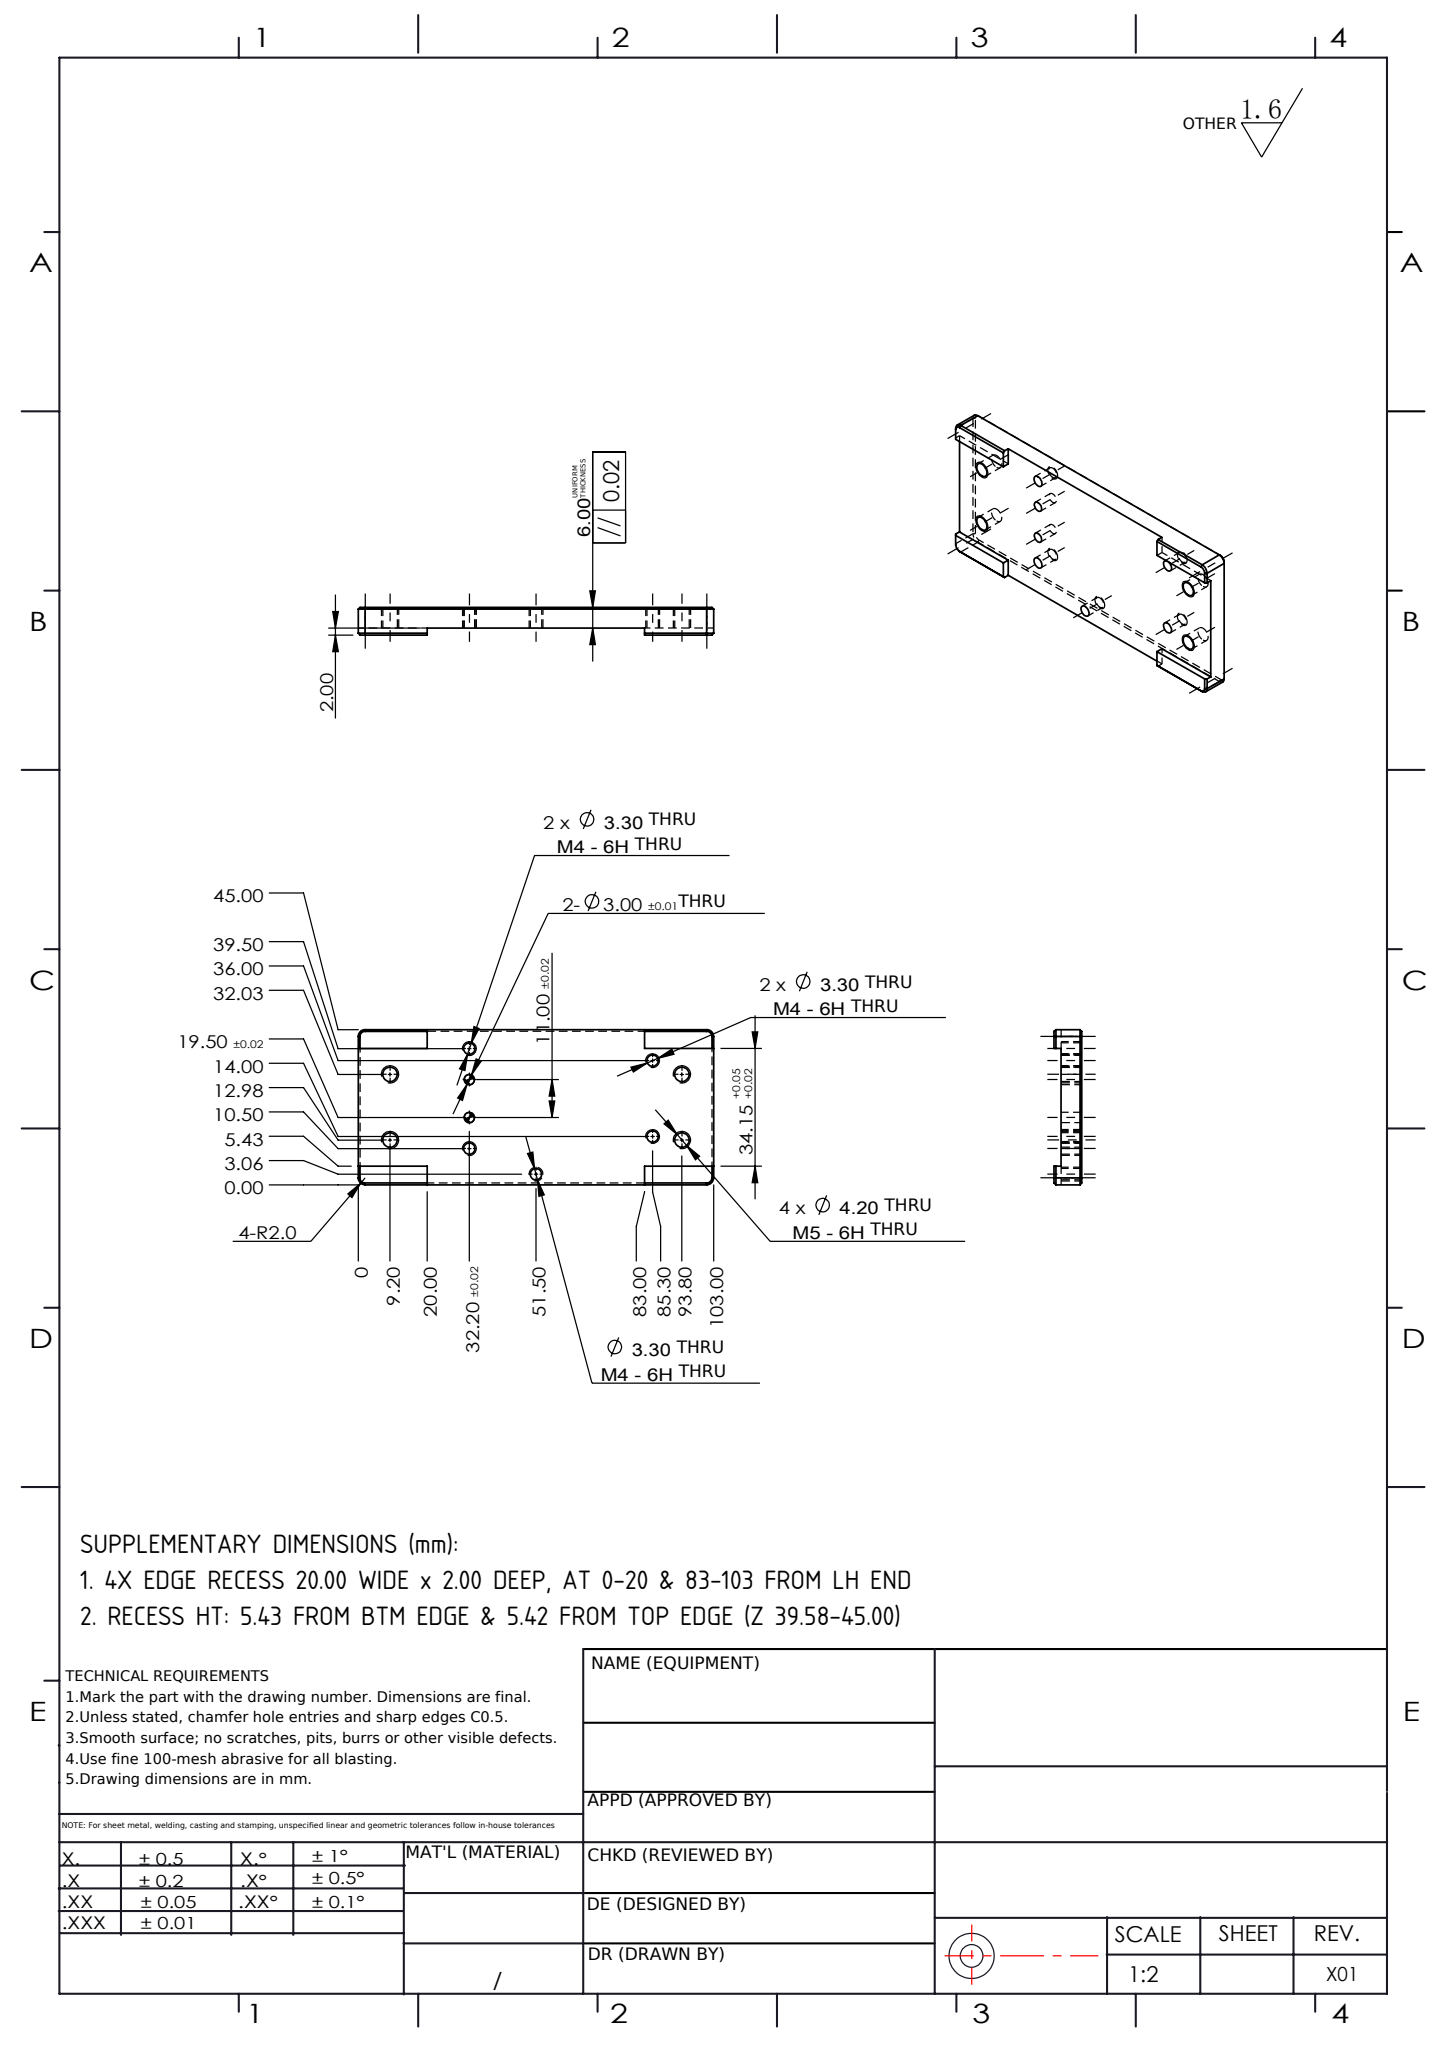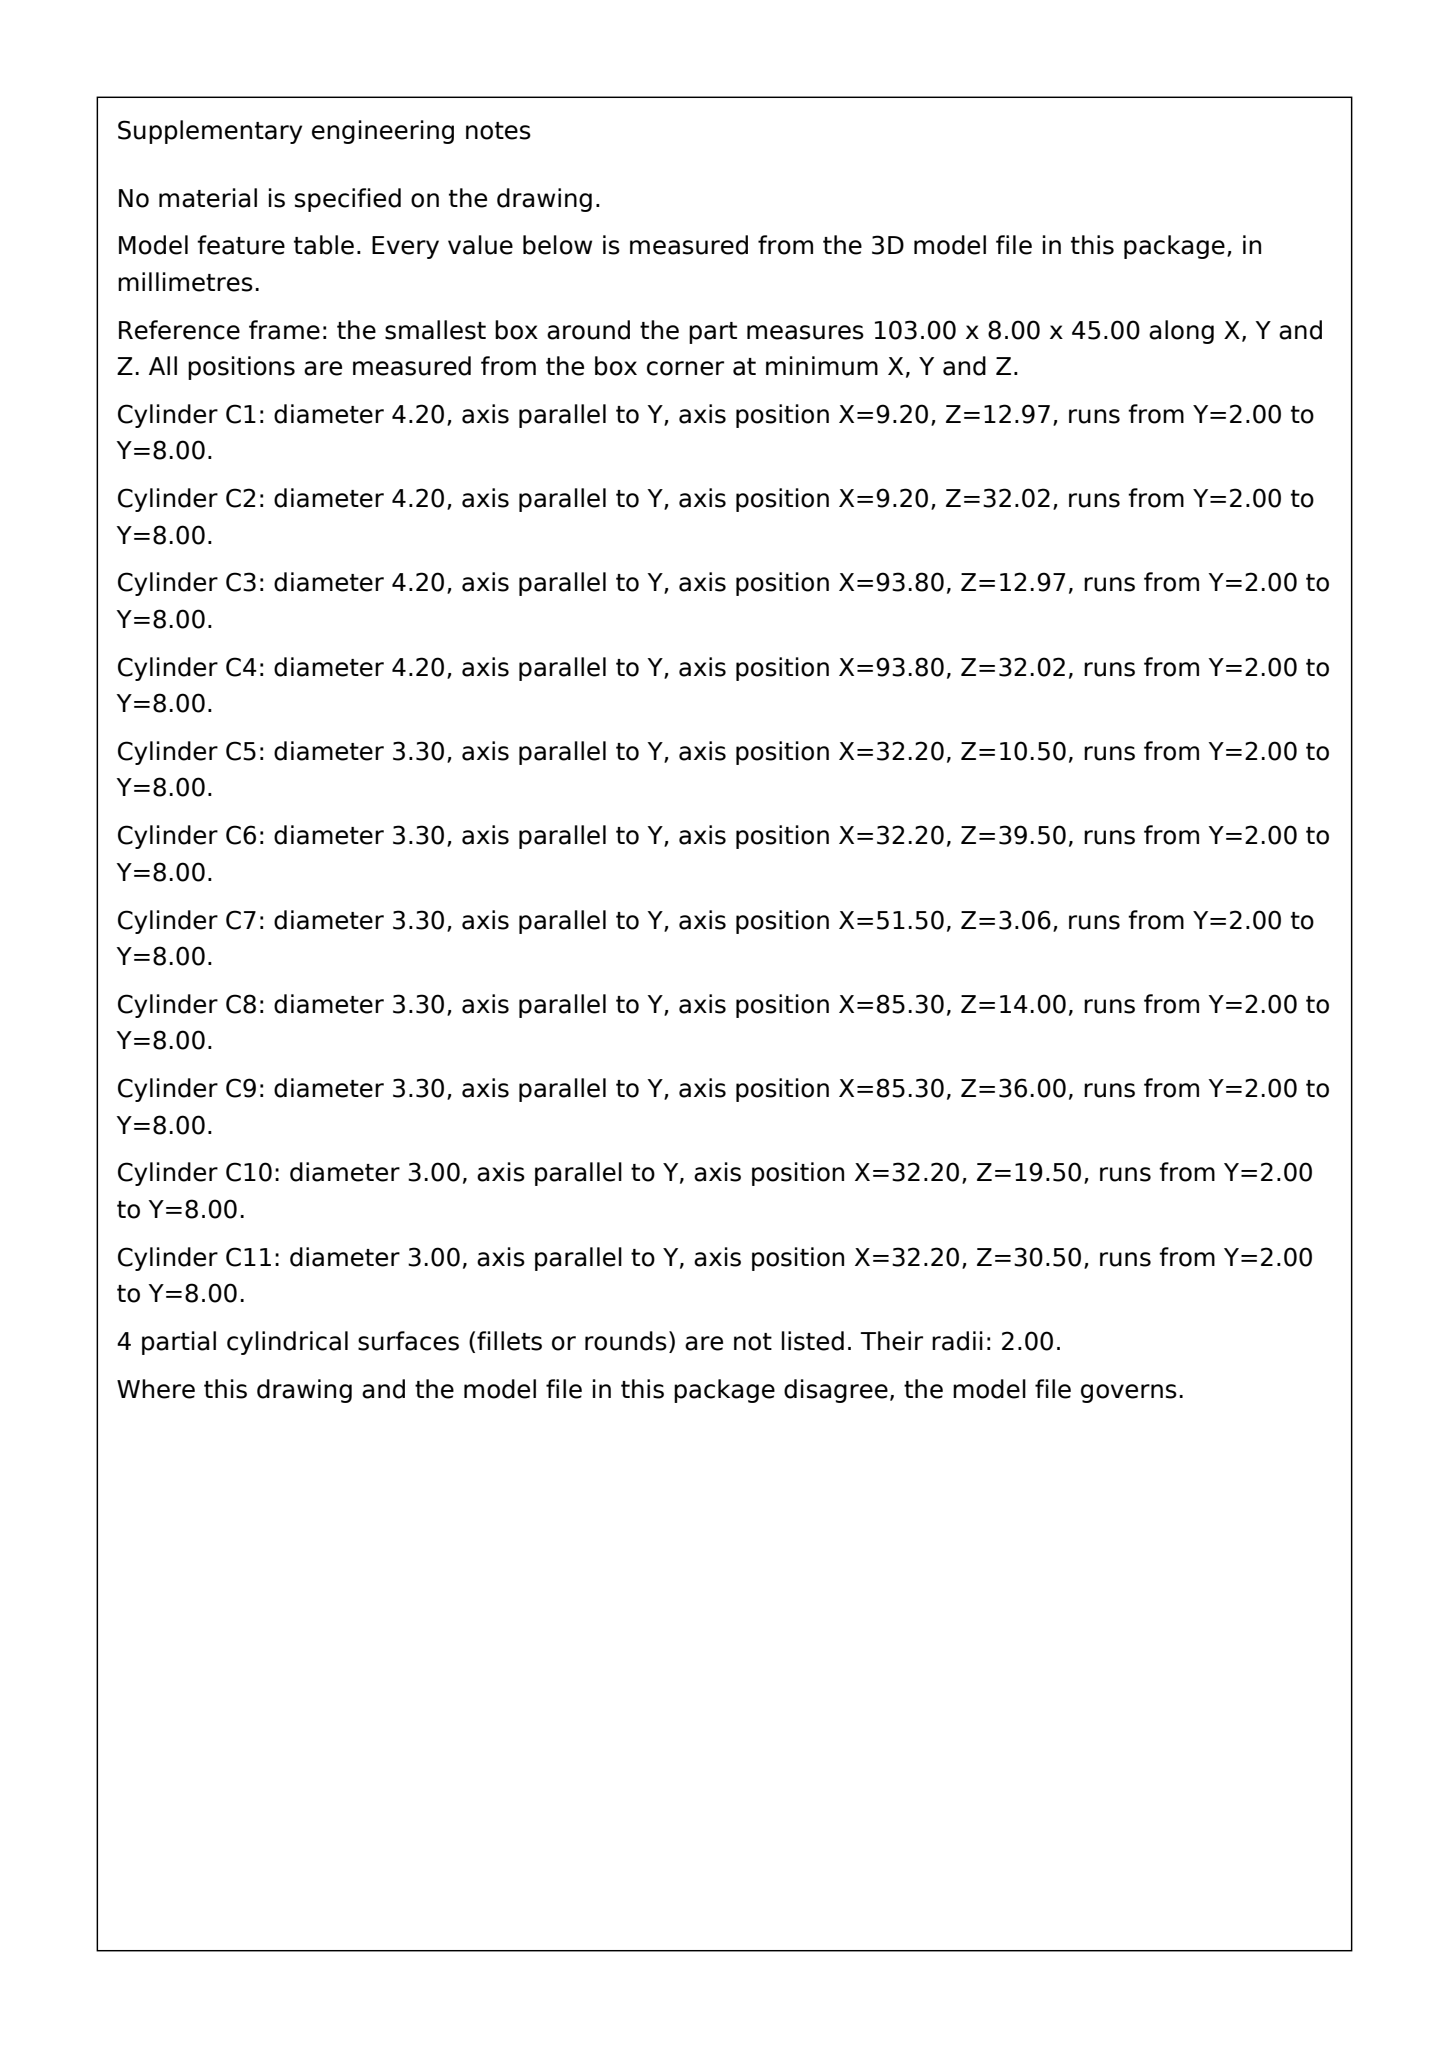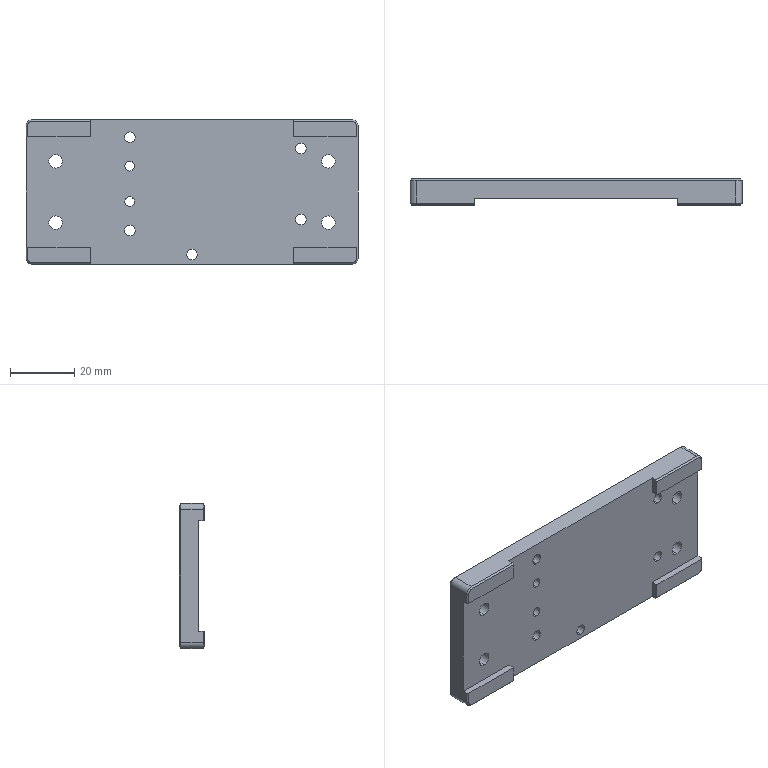Part | SolidWorks | mm | 1 solid | 64 faces | box 103 x 8 x 45 mm | volume 27928 mm3 | plane 30 | cylinder 26 | cone 8 | commonest cylinder face diameters 3.3 x10 4.2 x8 3 x4 4 x4
build123d program:
from build123d import *

# Parameters (mm, degrees)
SKETCH1_W                = 103
SKETCH1_H                = 45
BOSS_EXTRUDE1_DEPTH      = 8
SKETCH2_W                = 103
SKETCH2_H                = 34.15
CUT_EXTRUDE1_DEPTH       = 2
SKETCH3_W                = 63
SKETCH3_H                = 45
CUT_EXTRUDE2_DEPTH       = 2
M4_TAPPED_HOLE1_D        = 3.3
M5_TAPPED_HOLE1_D        = 4.2
FILLET1_R                = 2
M4_TAPPED_HOLE2_D        = 3.3
M4_TAPPED_HOLE3_D        = 3.3
F_3_0_3_DIAMETER_HOLE1_D = 3
CHAMFER1_SIZE            = 0.5


with BuildPart() as part:
    # Sketch1 → Boss-Extrude1 (new body)
    with BuildSketch(Plane(origin=(0, 0, 0), x_dir=(1, 0, 0), z_dir=(0, 1, 0))):
        Rectangle(SKETCH1_W, SKETCH1_H)
    extrude(amount=BOSS_EXTRUDE1_DEPTH)

    # Sketch2 → Cut-Extrude1 (cut)
    with BuildSketch(Plane.XZ):
        Rectangle(SKETCH2_W, SKETCH2_H)
    extrude(amount=-CUT_EXTRUDE1_DEPTH, mode=Mode.SUBTRACT)

    # Sketch3 → Cut-Extrude2 (cut)
    with BuildSketch(Plane.XZ):
        Rectangle(SKETCH3_W, SKETCH3_H)
    extrude(amount=-CUT_EXTRUDE2_DEPTH, mode=Mode.SUBTRACT)

    # M4 Tapped Hole1 (through all)
    with Locations(Plane(origin=(0, 8, 0), x_dir=(1, 0, 0), z_dir=(0, 1, 0))):
        with Locations((0, 19.436)):
            Hole(M4_TAPPED_HOLE1_D / 2)

    # M5 Tapped Hole1 (through all)
    with Locations(Plane(origin=(0, 2, 0), x_dir=(-1, 0, 0), z_dir=(0, -1, 0))):
        with Locations((-42.3, -9.525), (-42.3, 9.525), (42.3, -9.525), (42.3, 9.525)):
            Hole(M5_TAPPED_HOLE1_D / 2)

    # Fillet1
    fillet1_edges = [part.edges().sort_by_distance(p)[0] for p in [
        (51.5, 4, 22.5),
        (-51.5, 4, 22.5),
        (-51.5, 4, -22.5),
        (51.5, 4, -22.5),
    ]]
    fillet(fillet1_edges, radius=FILLET1_R)

    # M4 Tapped Hole2 (through all)
    with Locations(Plane(origin=(0, 8, 0), x_dir=(1, 0, 0), z_dir=(0, 1, 0))):
        with Locations((33.8, 8.5), (33.8, -13.5)):
            Hole(M4_TAPPED_HOLE2_D / 2)

    # M4 Tapped Hole3 (through all)
    with Locations(Plane(origin=(0, 8, 0), x_dir=(1, 0, 0), z_dir=(0, 1, 0))):
        with Locations((-19.3, -17), (-19.3, 12)):
            Hole(M4_TAPPED_HOLE3_D / 2)

    # 3.0 _3_ Diameter Hole1 (through all)
    with Locations(Plane(origin=(0, 8, 0), x_dir=(1, 0, 0), z_dir=(0, 1, 0))):
        with Locations((-19.3, -8), (-19.3, 3)):
            Hole(F_3_0_3_DIAMETER_HOLE1_D / 2)

    # Chamfer1
    chamfer1_edges = [part.edges().sort_by_distance(p)[0] for p in [
        (-50.914, 0, 21.914),
        (51.5, 0, -18.788),
        (-51.5, 0, 18.788),
        (40.5, 0, 22.5),
        (-40.5, 0, -22.5),
        (-51.5, 0, -18.788),
        (-51.5, 8, 0),
        (-50.914, 0, -21.914),
        (0, 8, -22.5),
        (40.5, 0, -22.5),
        (51.5, 8, 0),
        (0, 8, 22.5),
        (-50.914, 8, 21.914),
        (50.914, 8, 21.914),
        (50.914, 8, -21.914),
        (-50.914, 8, -21.914),
        (50.914, 0, -21.914),
        (51.5, 0, 18.788),
        (50.914, 0, 21.914),
        (-40.5, 0, 22.5),
    ]]
    chamfer(chamfer1_edges, length=CHAMFER1_SIZE)


solid = part.part